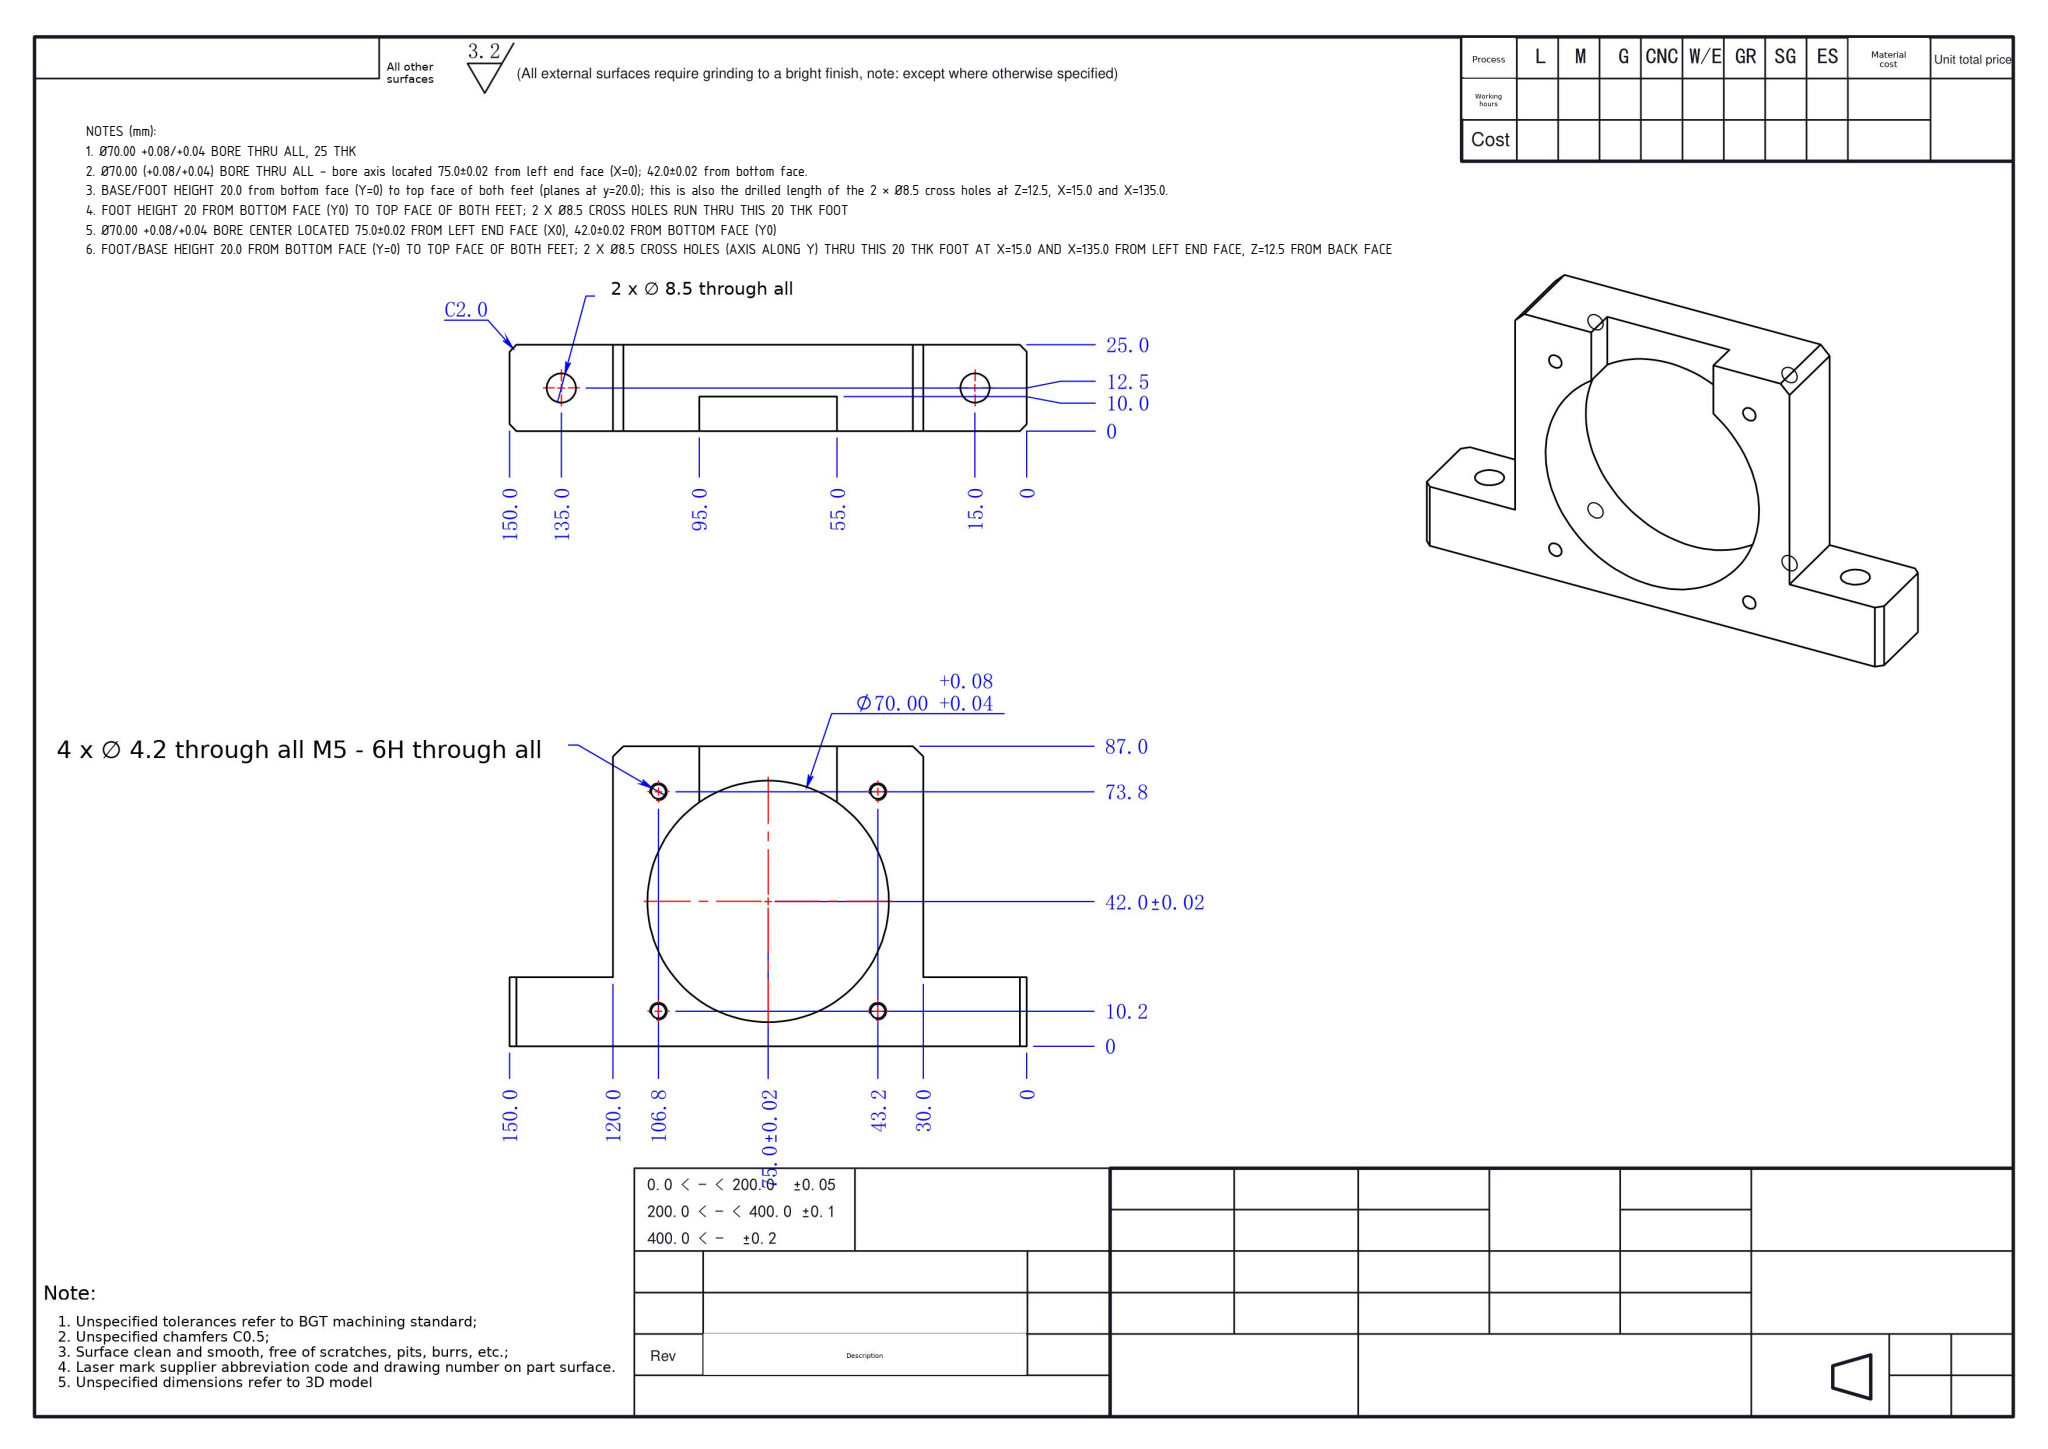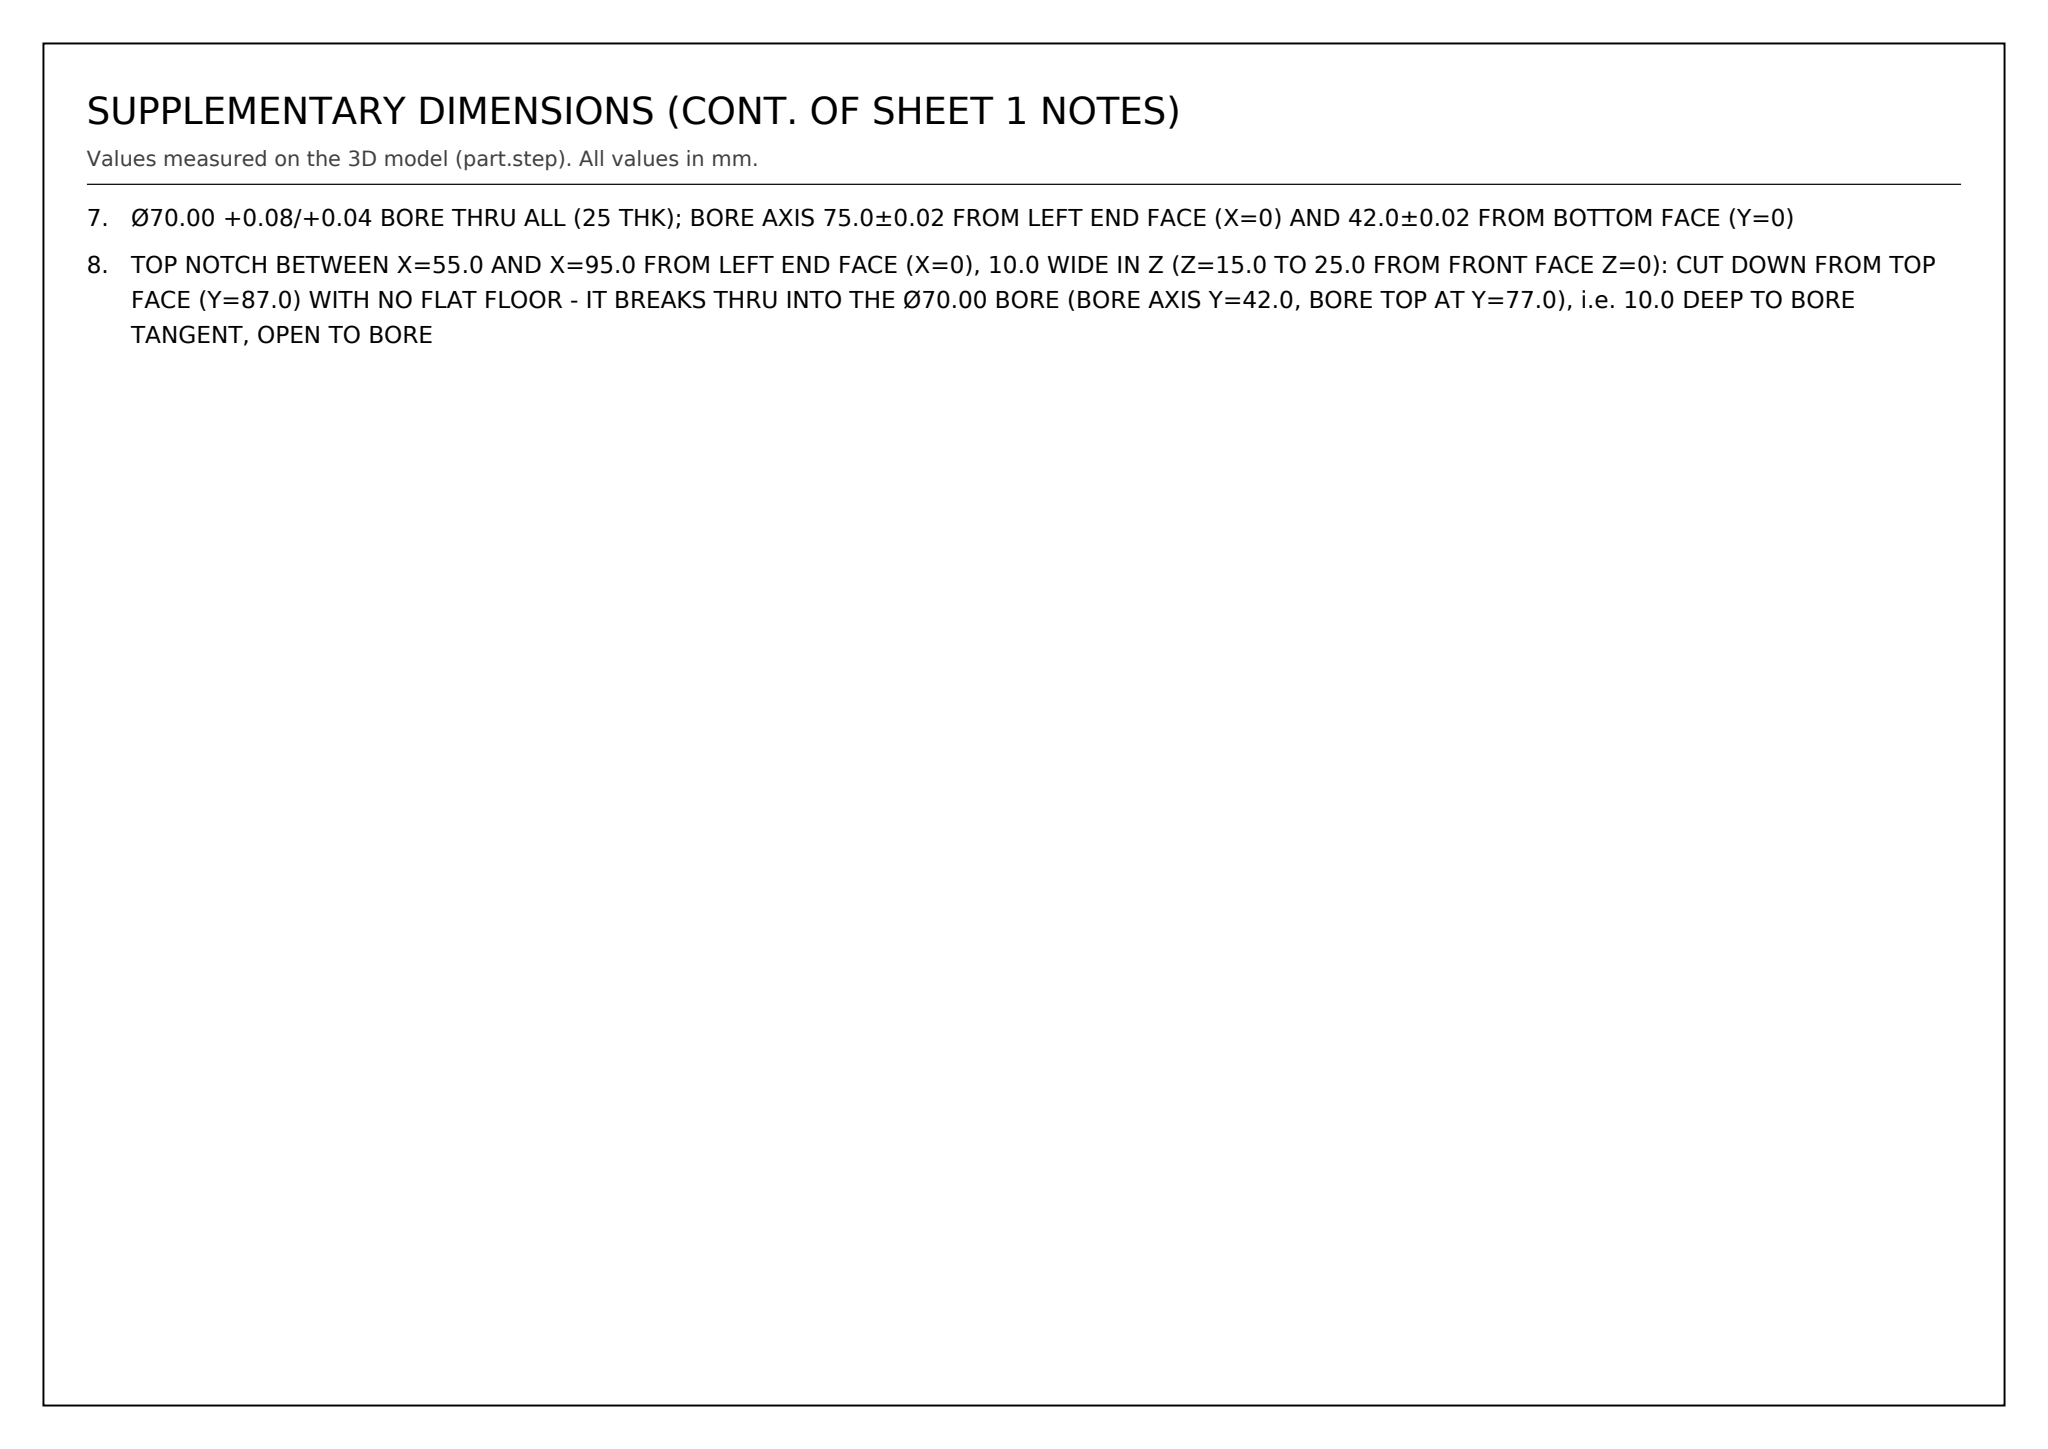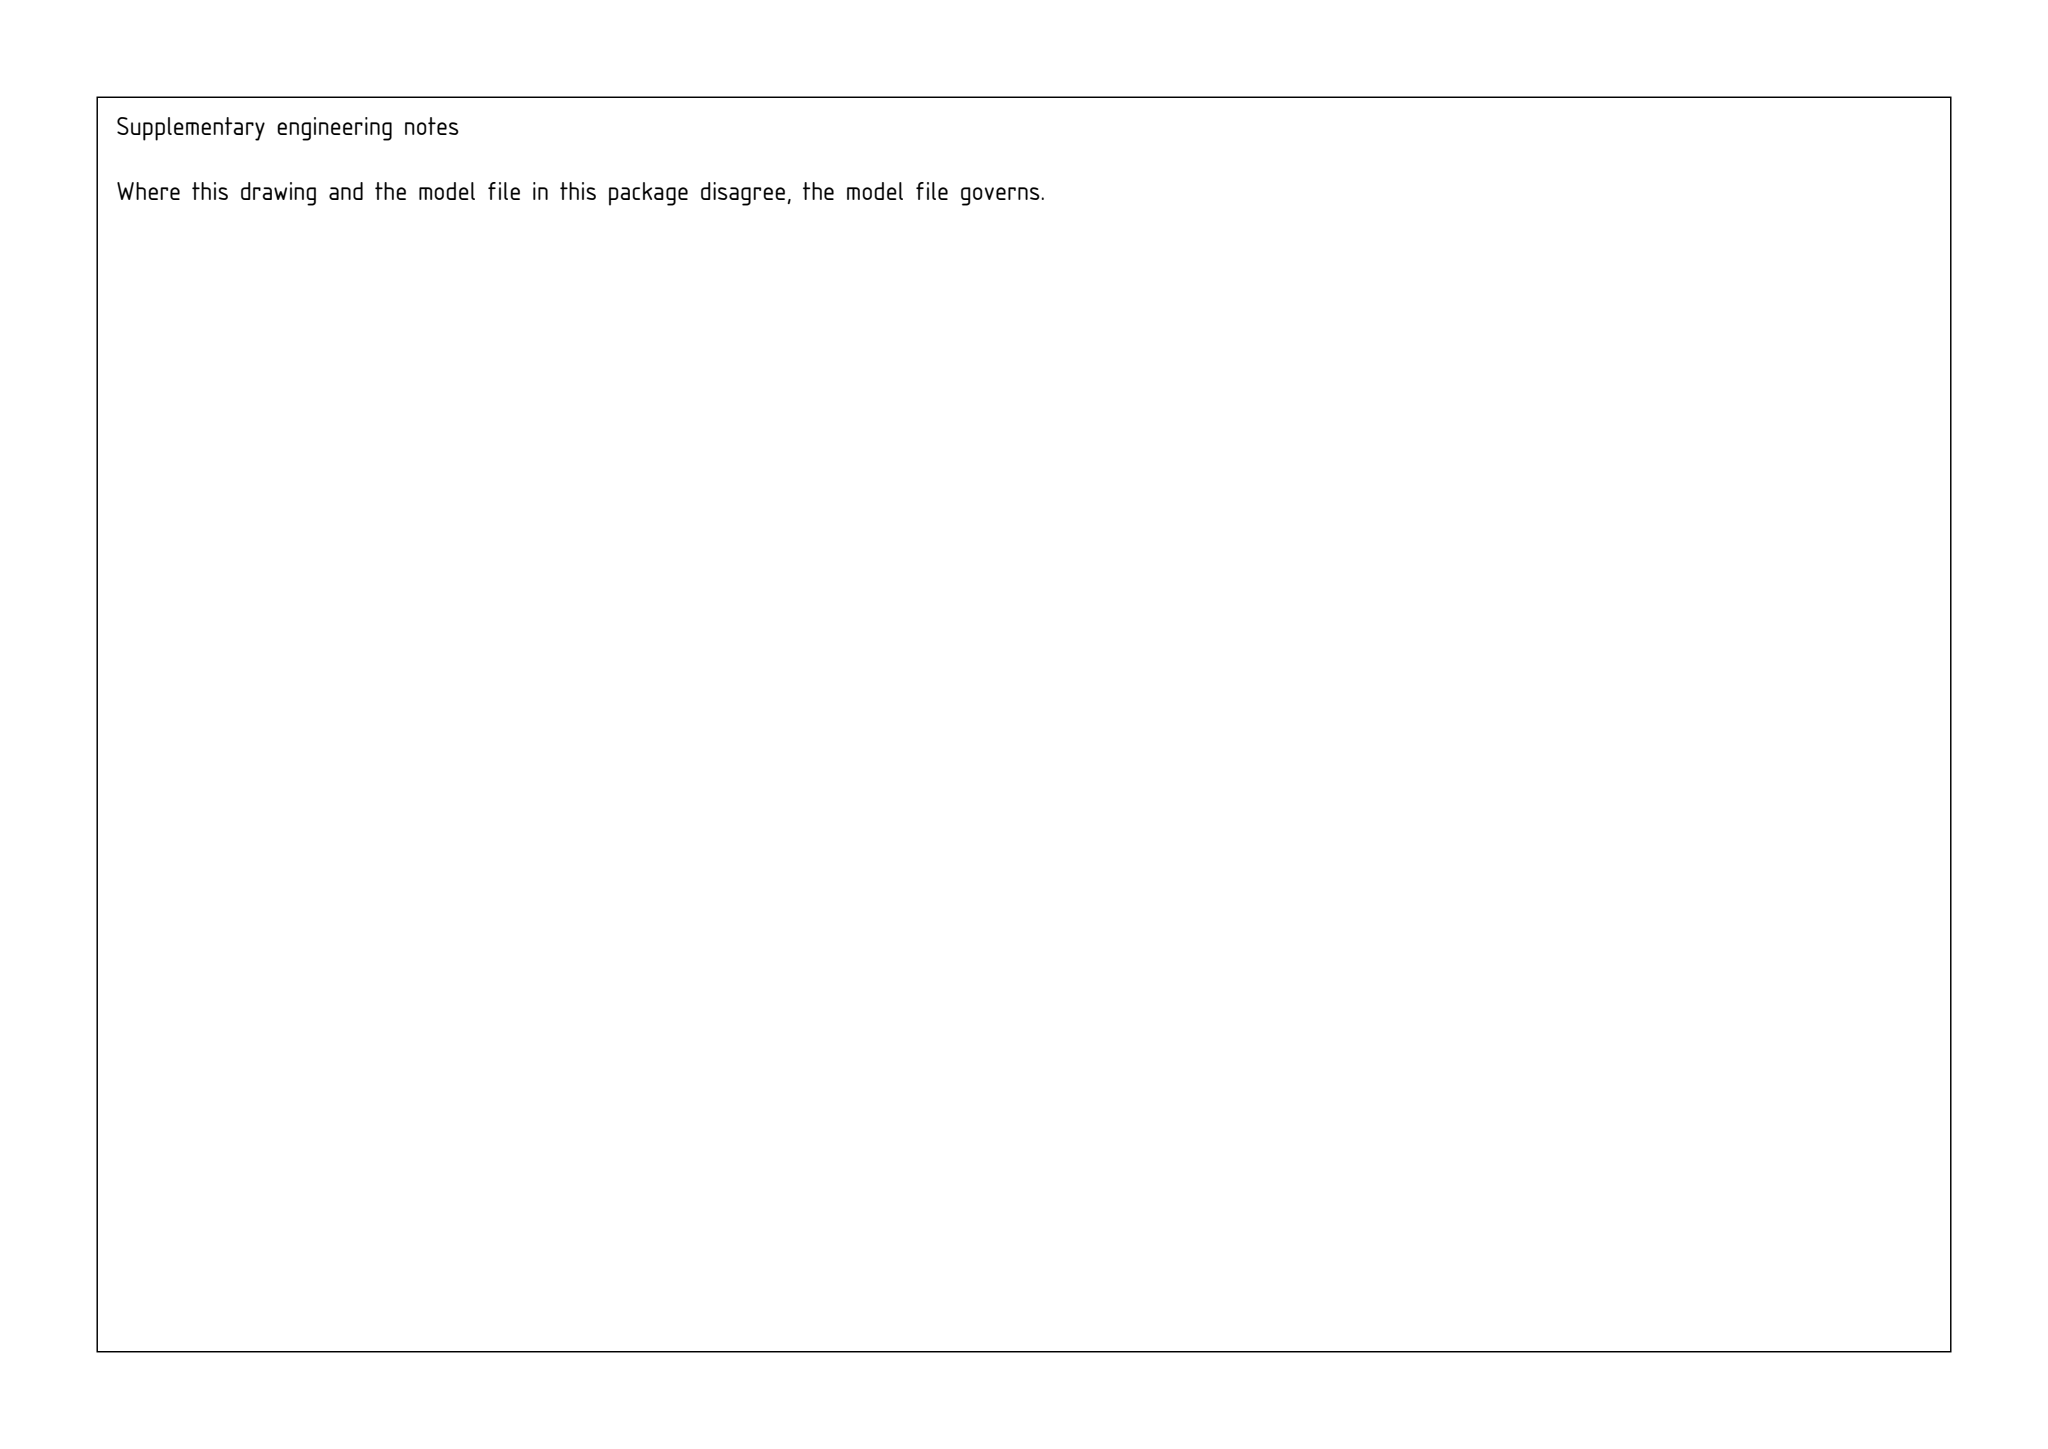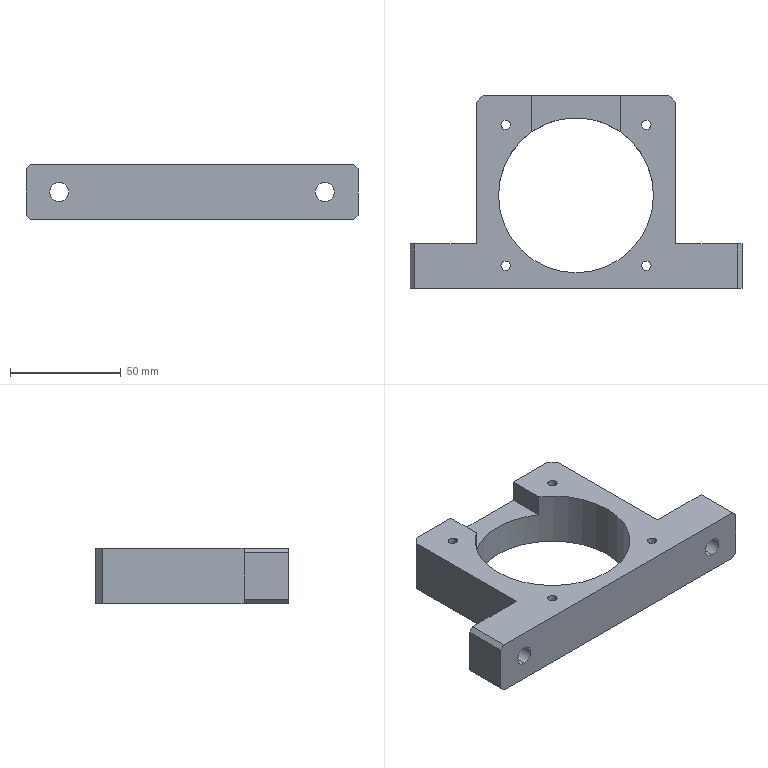Part | SolidWorks | mm | 1 solid | 33 faces | box 150 x 87 x 25 mm | volume 120694 mm3 | plane 19 | cylinder 14 | commonest cylinder face diameters 4.2 x8 8.5 x4 70 x2
Drawing notes:
Ø70.00 +0.08/+0.04 BORE THRU ALL, 25 THK | from the solid: cylinder dia 70, axis z at (75.0, 42.0), length 25.0 = full Z extent of bbox (25.0)
Ø70.00 (+0.08/+0.04) BORE THRU ALL - bore axis located 75.0±0.02 from left end face (X=0); 42.0±0.02 from bottom face. | from the solid: cylinder dia 70.0, axis z, position [75.0, 42.0], length 25.0
BASE/FOOT HEIGHT 20.0 from bottom face (Y=0) to top face of both feet (planes at y=20.0); this is also the drilled length of the 2 × Ø8.5 cross holes at Z=12.5, X=15.0 and X=135.0. | from the solid: axis_planes y=20.0 (count 2); cylinders dia 8.5, axis y, pos [15.0, z12.5] and [135.0, z12.5], length 20.0
FOOT HEIGHT 20 FROM BOTTOM FACE (Y0) TO TOP FACE OF BOTH FEET; 2 X Ø8.5 CROSS HOLES RUN THRU THIS 20 THK FOOT | from the solid: axis_planes y=20.0 (count 2); cylinders dia 8.5 axis y length 20.0 at x=15.0 and x=135.0, z=12.5
Ø70.00 +0.08/+0.04 BORE CENTER LOCATED 75.0±0.02 FROM LEFT END FACE (X0), 42.0±0.02 FROM BOTTOM FACE (Y0) | from the solid: cylinders [70.0, axis z, pos [75.0, 42.0], length 25.0]
FOOT/BASE HEIGHT 20.0 FROM BOTTOM FACE (Y=0) TO TOP FACE OF BOTH FEET; 2 X Ø8.5 CROSS HOLES (AXIS ALONG Y) THRU THIS 20 THK FOOT AT X=15.0 AND X=135.0 FROM LEFT END FACE, Z=12.5 FROM BACK FACE | from the solid: axis_planes y=0.0 and y=20.0; cylinders [8.5,"y",[15.0,null,12.5],20.0] and [8.5,"y",[135.0,null,12.5],20.0]
Ø70.00 +0.08/+0.04 BORE THRU ALL (25 THK); BORE AXIS 75.0±0.02 FROM LEFT END FACE (X=0) AND 42.0±0.02 FROM BOTTOM FACE (Y=0) | from the solid: cylinder [70.0,"z",[75.0,42.0,null],25.0]; bbox_xyz 150.0 x 87.0 x 25.0
TOP NOTCH BETWEEN X=55.0 AND X=95.0 FROM LEFT END FACE (X=0), 10.0 WIDE IN Z (Z=15.0 TO 25.0 FROM FRONT FACE Z=0): CUT DOWN FROM TOP FACE (Y=87.0) WITH NO FLAT FLOOR - IT BREAKS THRU INTO THE Ø70.00 BORE (BORE AXIS Y=42.0, BORE TOP AT Y=77.0), i.e. 10.0 DEEP TO BORE TANGENT, OPEN TO BORE | from the solid: axis_planes y only at 0.0 / 20.0 / 87.0 (no intermediate floor plane); x planes at 55.0 and 95.0; z planes at 15.0 and 25.0; cylinder dia 70.0 axis z at [75.0, 42.0] so bore top = 42.0+35.0 = 77.0 < 87.0 top face